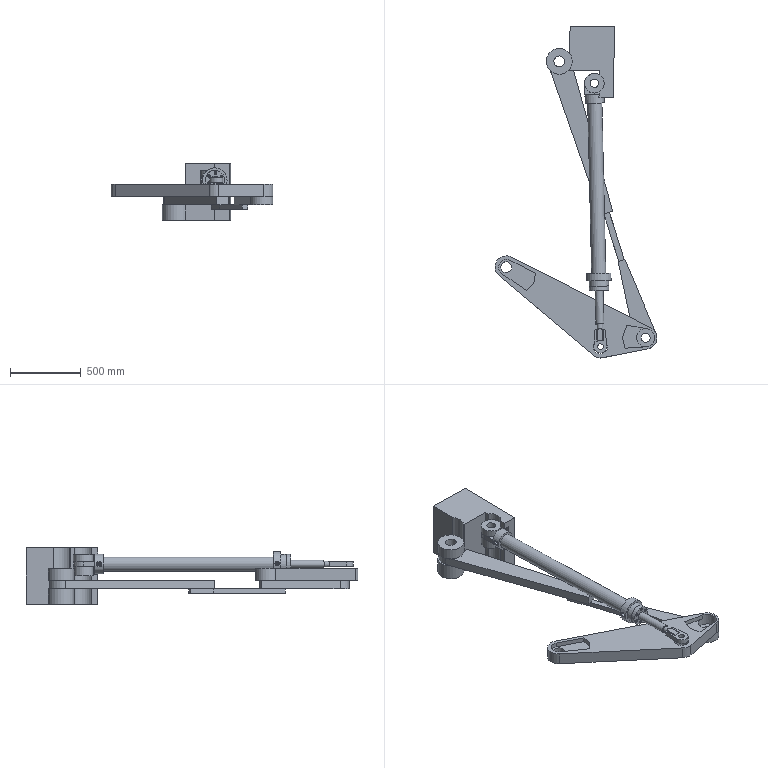Assembly | NX | mm | 10 component files | 10 solids | 200 faces | box 1141.39 x 2338.78 x 400 mm | volume 97661417 mm3 | plane 124 | cylinder 75 | cone 1 | commonest cylinder face diameters 20 x12 40 x6 12 x6 138.98 x5 160 x5 136 x4 80 x4 182.323 x4
Bill of materials:
unnamed part 1 | 1 |  | Stepped cylindrical boss with a flat tab sticking out sideways. The tab has a rounded end and one round through hole. A smaller hollow cylindrical spigot sticks out from the larger cylinder.
unnamed part 2 | 1 |  | Stepped cylindrical spacer or bushing with a central through bore. It has a large center collar with a smaller hub on each side, and the two hubs have different diameters.
unnamed part 3 | 1 |  | Stepped tubular sleeve. A larger-diameter middle section sits between two smaller-diameter hollow ends, with a through bore along the axis.
unnamed part 4 | 1 |  | Flat plate of constant thickness shaped like a fork or clevis. One end is rounded with a round through hole, and the other end splits into two prongs with an open rectangular slot between them.
unnamed part 5 | 1 |  | Flat annular disc or flange with a large central bore and six smaller through holes evenly spaced on a circle around it.
unnamed part 6 | 1 |  | Thin, flat, roughly triangular link plate that tapers along its length. It has one round hole near the narrow end and two holes near the wide end, one of them larger.
unnamed part 7 | 1 |  | Rectangular block with two ring-shaped lugs along one edge. Each lug has a round through hole, and the lugs sit at different heights and positions. The top face has a concave arc cut-out next to a lug.
unnamed part 8 | 1 |  | Long, slender, round shaft. Both ends step down to a smaller diameter, and one end has a flat-sided tip and a small groove or neck.
unnamed part 9 | 1 |  | Straight, plain round tube with a uniform hollow section and square-cut ends.
unnamed part 10 | 1 |  | Long, slender, flat arm with a round hole at each end. It is made of a long tapered segment and a short tapered segment, joined by a narrow neck that is offset in height.
Mates:
1. fix | 1 1 component
2. concentric | 3 1 | 1 1
3. concentric | 1 1 | 5 1
4. concentric | 7 1 | 5 1
5. concentric | 7 1 | 9 1
6. fix | frame 1 component
7. concentric | tri_arm 1 arc | tie_rod 1 edge
8. touch align | 6 1 face | hyd_cyl 1 face
9. touch align | 11 1 face | 6 1 face
10. center | 6 1 face | 6 1 face | 11 1 line
11. center | 11 1 line | 11 1 line | 6 1 face
12. touch align | 11 1 face | tri_arm 1 face
13. concentric | frame 1 edge | hyd_cyl 1 edge
14. concentric | tie_rod 1 arc | frame 1 edge
15. touch align | 6 1 face | hyd_cyl 1 face